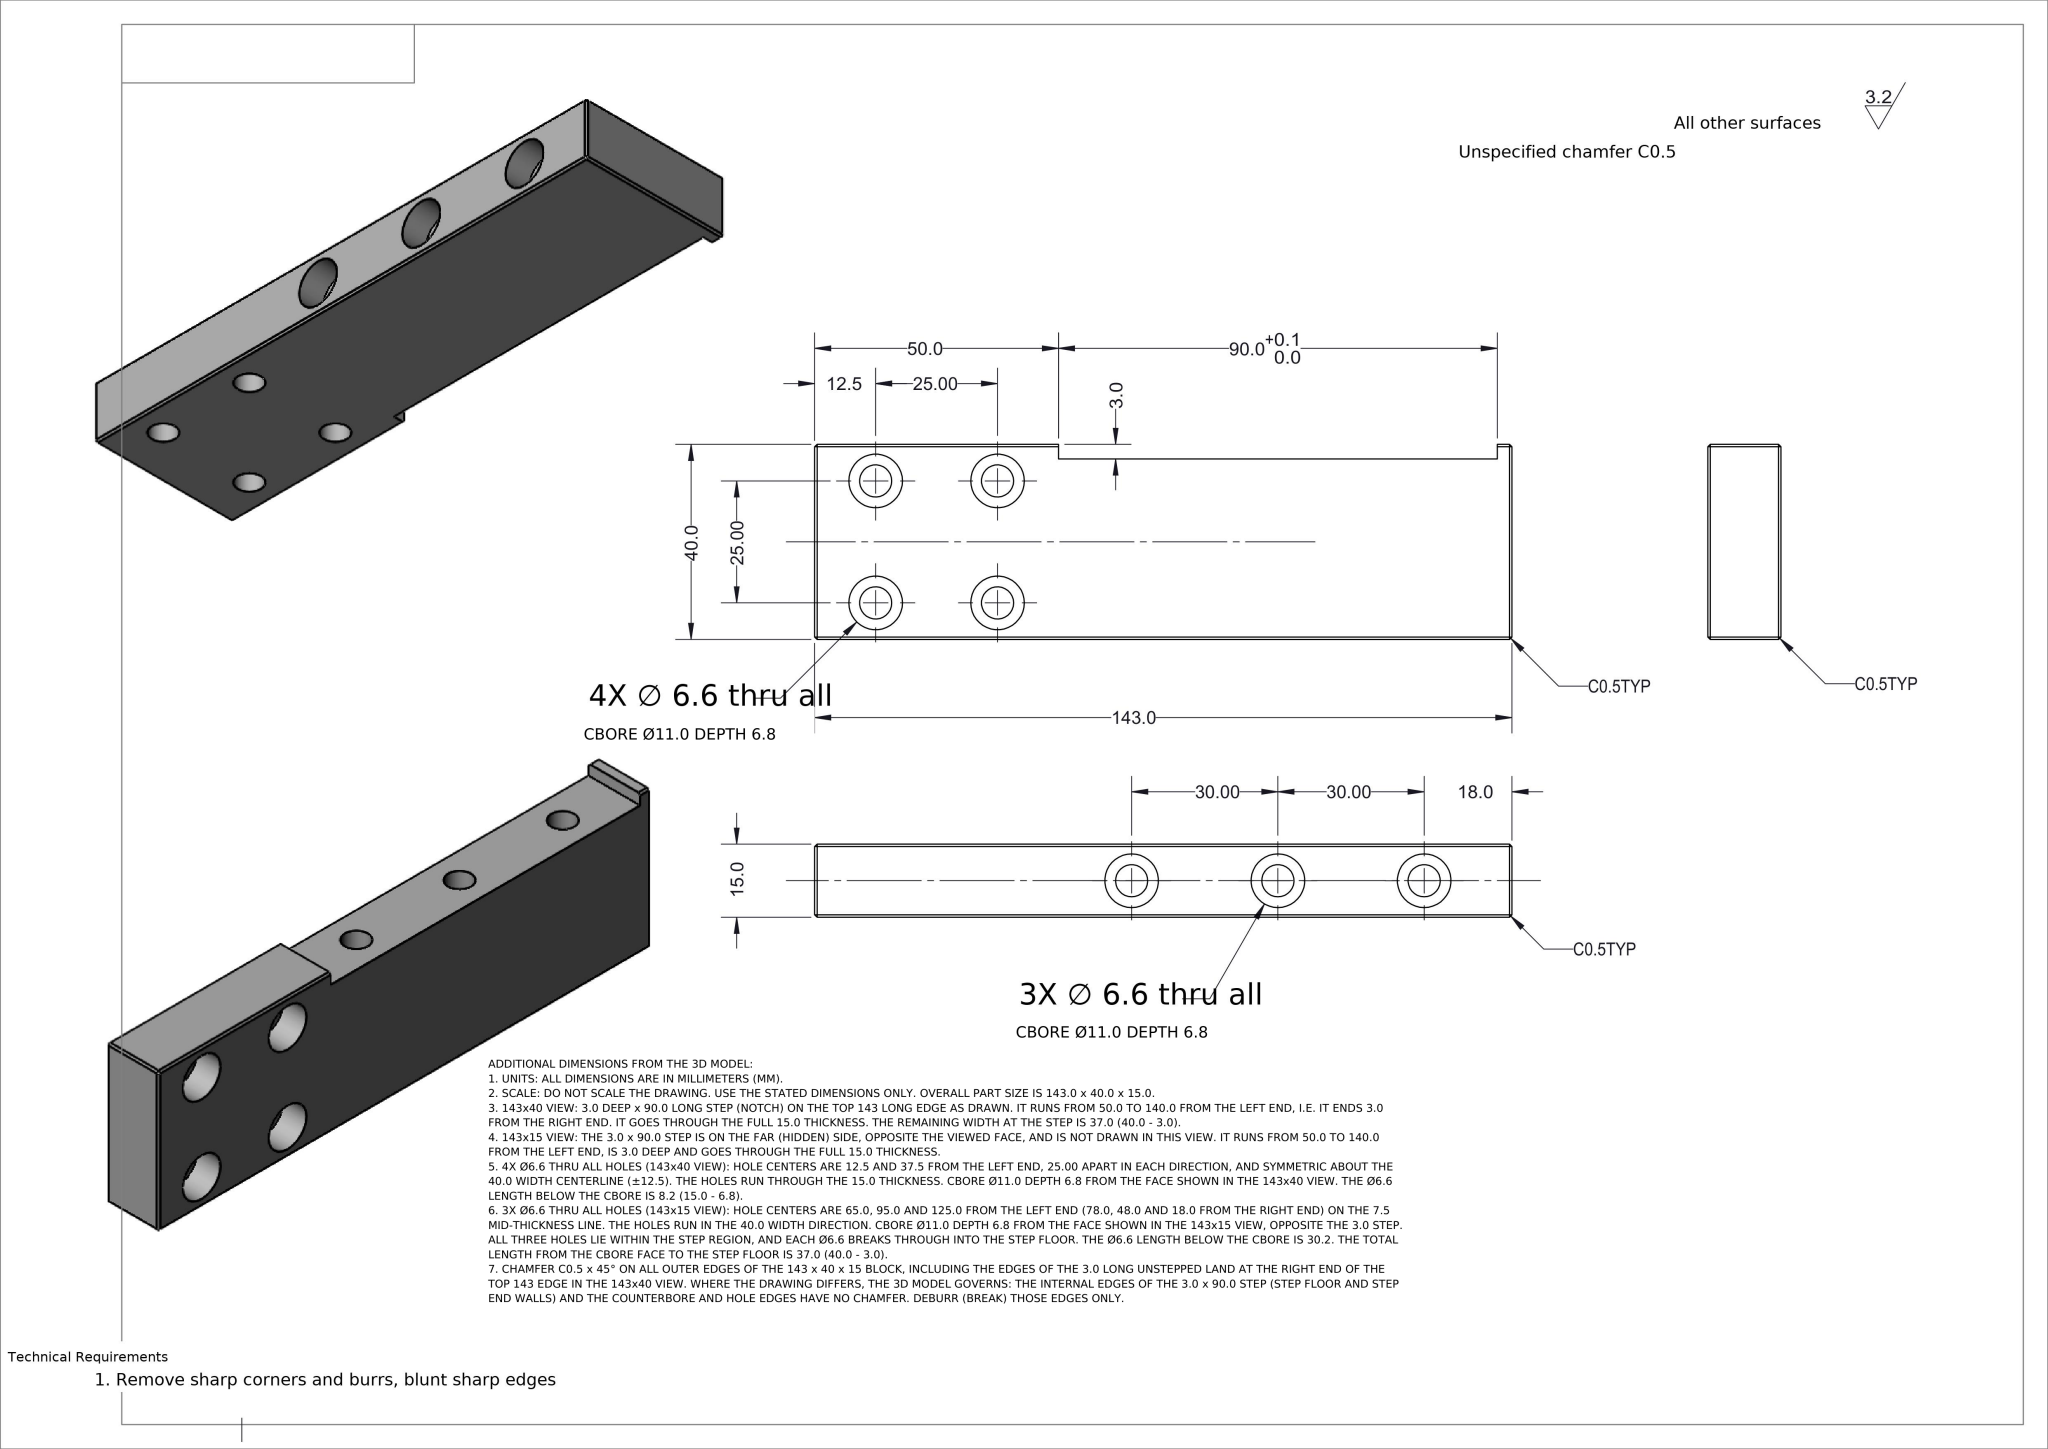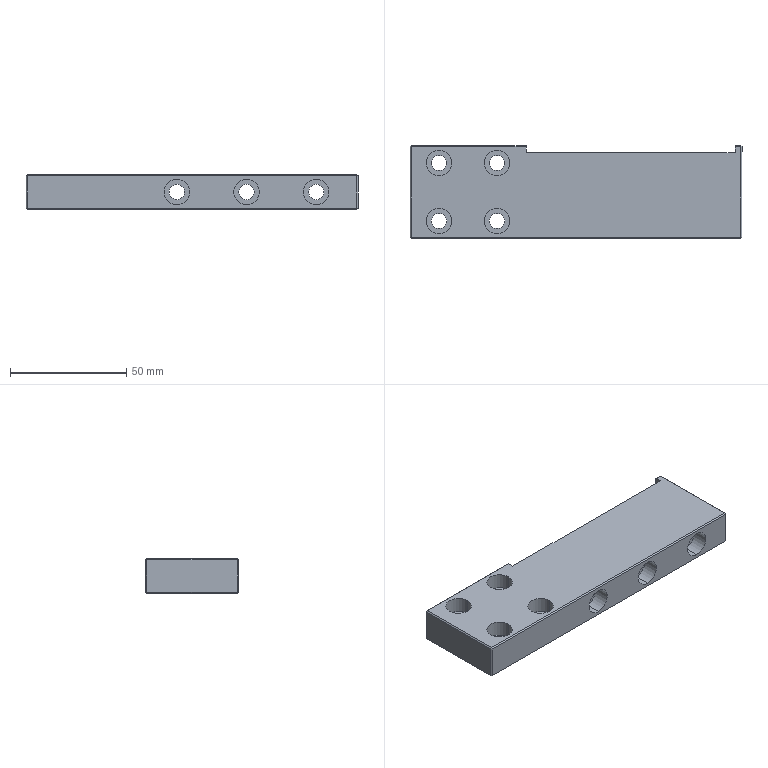Part | NX | mm | 1 solid | 67 faces | box 143 x 40 x 15 mm | volume 72929 mm3 | plane 39 | cylinder 28 | commonest cylinder face diameters 11 x14 6.6 x14